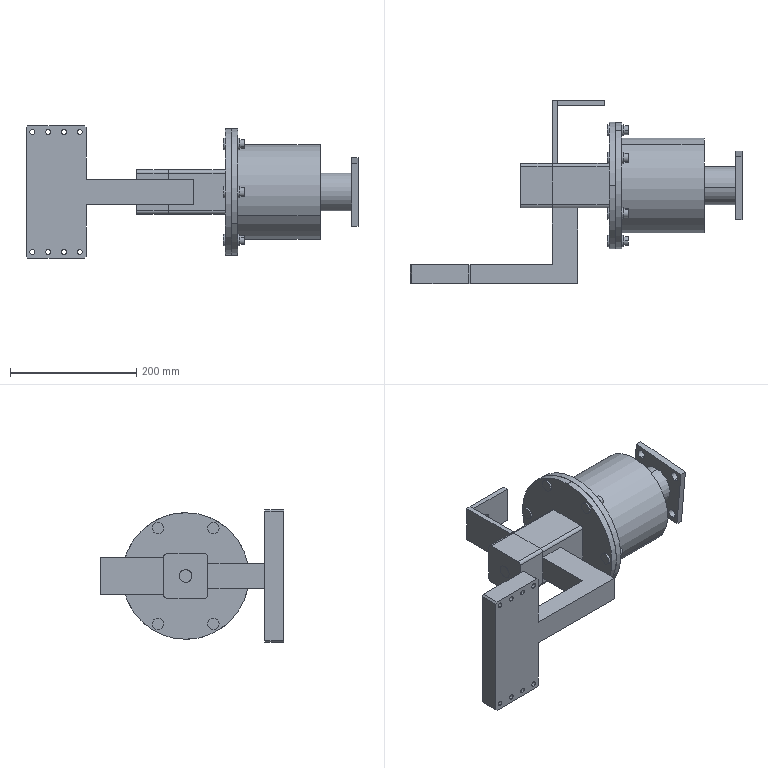Assembly | SolidWorks | mm | 20 component files | 40 solids | 384 faces | box 525 x 290 x 210 mm | volume 4267025 mm3 | cylinder 151 | plane 135 | torus 48 | cone 48 | sphere 2 | commonest cylinder face diameters 14 x58 18 x24 8 x16 10 x12 60 x10 20 x9 100 x6 200 x4
Bill of materials:
7mmNut | 6 |  | Plain annular ring: a short hollow cylinder with flat parallel faces and a rectangular cross-section.
7mmScrew | 6 |  | Solid cylindrical pin with a thin, larger-diameter head or collar at one end. Both ends are flat.
Arm4 | 1 |  | Multi-element bracket-like body. A rectangular plate with chamfered corners and two rows of four holes is joined by a rectangular-section bar with a bend to a circular flange. The flange has a central bore and a ring of bolt holes. There is also a rectangular block next to the flange and a thin L-shaped sheet section behind it.
ArmServoMotor | 1 |  | Rectangular block with rounded edges along one axis and one round through hole in the middle of the face that has the rounded corners.
ArmServoMotorAxis | 1 |  | Long solid cylindrical rod with a narrow rectangular rib or tab that projects radially along a short length at one end.
LowerCoupler | 1 |  | Cylindrical shaft or tube joining a larger-diameter disc at one end to a thin square plate at the other. The disc has a radial slot or notch. The plate has four corner holes and a hole near its center.
MiddleCoupler | 1 |  | Cylindrical disc with a small rectangular tab or boss projecting axially and off-center from one face. There is a straight step or slot feature across the other side.
UpperCoupler | 1 |  | Stepped cylinder: a smaller-diameter cylindrical section joined to a larger-diameter disc section. A straight slot runs across the whole end face of the larger section.
CouplerMountingPlate | 1 |  | Flanged cylindrical hub: a thick-walled cylinder with a central through bore and a thin circular flange at one end. The flange has six evenly spaced holes.
Rolling bearings 29412 GB 5859-94 | 1 |  | Annular, axisymmetric multi-body ring set: a wider outer ring, a narrower stepped inner ring with a central through-bore, and a single circumferential row of many small roller-like elements between them, set on an angle. The overall form looks like a tapered roller bearing (cup, cone and rollers), but this is inferred from shape only.
Mates:
1. concentric | Arm4-1 face at (-114.36, 70.663, 0) dir (1, 0, 0) r 10 | ArmServoMotorAssembly-1/ArmServoMotorAxis-1 face at (-34.359, 70.663, 0) dir (1, 0, 0) r 10
2. coincident | Arm4-1 face at (15.641, -84.337, -20) dir (-1, 0, 0) | ArmServoMotorAssembly-1/ArmServoMotor-1 face at (15.641, 35.663, -35) dir (1, 0, 0)
3. concentric | ArmServoMotorAssembly-1/ArmServoMotorAxis-1 face at (-34.359, 70.663, 0) dir (1, 0, 0) r 10 | CouplerAssembly-1/UpperCoupler-1 face at (105.641, 70.663, 0) dir (-1, 0, 0) r 10
4. coincident | ArmServoMotorAssembly-1/ArmServoMotorAxis-1 face at (105.641, 70.663, 0) dir (1, 0, 0) | CouplerAssembly-1/UpperCoupler-1 face at (105.641, 70.663, 0) dir (-1, 0, 0)
5. coincident | ArmServoMotorAssembly-1/ArmServoMotorAxis-1 face at (105.641, 68.852, -13.218) dir (0, -0.9959, -0.09053) | CouplerAssembly-1/UpperCoupler-1 face at (105.641, 68.852, -13.218) dir (0, 0.9959, 0.09053)
6. concentric | CouplerAssembly-1/LowerCoupler-1 face at (305.641, 70.663, 0) dir (-1, 0, 0) r 30 | self-aligning thrust roller bearings gb-1 face at (288.545, 70.663, 0) dir (1, 0, 0) r 31.5
7. coincident | CouplerAssembly-1/LowerCoupler-1 face at (205.641, 70.663, 0) dir (1, 0, 0) | self-aligning thrust roller bearings gb-1 face at (205.641, 72.046, -31.47) dir (-1, 0, 0)
8. concentric | CouplerAssembly-1/LowerCoupler-1 face at (205.641, 70.663, 0) dir (-1, 0, 0) r 50 | CouplerMountingPlate-2 face at (247.641, 70.663, 0) dir (-1, 0, 0) r 65
9. coincident | self-aligning thrust roller bearings gb-1 face at (247.641, 70.663, 0) dir (1, 0, 0) | CouplerMountingPlate-2 face at (247.641, 70.663, 0) dir (-1, 0, 0)
10. concentric | Arm4-1 face at (-114.36, 158.163, 0) dir (1, 0, 0) r 7 | CouplerMountingPlate-2 face at (115.641, 158.163, 0) dir (1, 0, 0) r 7
11. concentric | Arm4-1 face at (-114.36, 158.163, 0) dir (1, 0, 0) r 7 | 7mmScrew-7 face at (135.641, 158.163, 0) dir (-1, 0, 0) r 7
12. coincident | Arm4-1 face at (105.641, 70.663, 0) dir (-1, 0, 0) | 7mmScrew-7 face at (105.641, 158.163, 0) dir (1, 0, 0)
13. concentric | 7mmScrew-7 face at (135.641, 158.163, 0) dir (-1, 0, 0) r 7 | 7mmNut-2 face at (125.64, 158.163, 0) dir (1, 0, 0) r 7
14. coincident | CouplerMountingPlate-2 face at (125.641, 70.663, 0) dir (1, 0, 0) | 7mmNut-2 face at (125.641, 158.163, 0) dir (-1, 0, 0)
15. coincident | Arm4-1 face at (15.641, 35.663, 35) dir (0, 0, 1) | ArmServoMotorAssembly-1/ArmServoMotor-1 face at (15.641, 105.663, 35) dir (0, 0, 1)
16. concentric | ArmServoMotor-1 face at (-9.163, 3.757, -25.001) dir (0, 0, 1) r 10 | ArmServoMotorAxis-1 face at (-9.163, 3.757, -25) dir (0, 0, 1) r 10
17. coincident | ArmServoMotor-1 face at (25.837, -31.243, -25) dir (0, 0, -1) | ArmServoMotorAxis-1 face at (-9.163, 3.757, -25) dir (0, 0, -1)
18. coincident | UpperCoupler-1 face at (-68.197, 12.225, -10) dir (0, -1, 0) | MiddleCoupler-1 face at (31.804, 12.225, -10) dir (0, 1, 0)
19. concentric | UpperCoupler-1 face at (-18.196, 2.225, 0) dir (0, 0, -1) r 50 | MiddleCoupler-1 face at (-18.196, 2.225, -30) dir (0, 0, -1) r 50
20. coincident | UpperCoupler-1 face at (-68.197, -7.775, -10) dir (0, 0, -1) | MiddleCoupler-1 face at (-68.196, -7.775, -10) dir (0, 0, 1)
21. concentric | MiddleCoupler-1 face at (-18.196, 2.225, -30) dir (0, 0, -1) r 50 | LowerCoupler-1 face at (-18.196, 2.225, -90) dir (0, 0, 1) r 50
22. coincident | MiddleCoupler-1 face at (-28.196, -47.775, -80) dir (-1, 0, 0) | LowerCoupler-1 face at (-28.196, 52.226, -80) dir (1, 0, 0)
23. coincident | MiddleCoupler-1 face at (-18.196, 2.225, -60) dir (0, 0, -1) | LowerCoupler-1 face at (-18.196, 2.225, -60) dir (0, 0, 1)